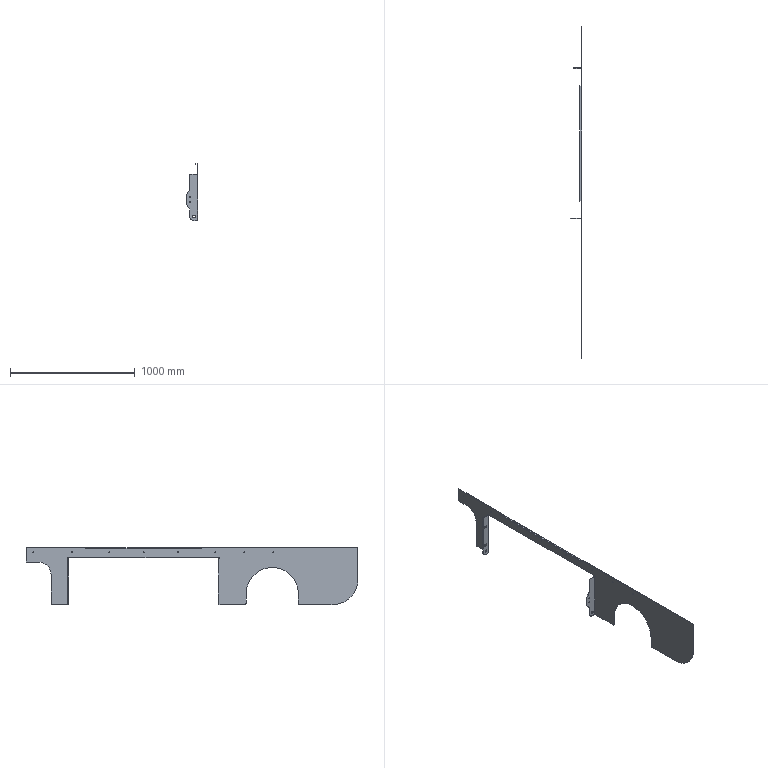Component | SolidWorks | BodySidePlate,Right-1 | 1 solid | 97 faces | volume 3195637 mm3 | plane 55 | cylinder 42 | commonest cylinder face diameters 7.2 x16 10.2 x4 20.2 x4 10 x4 20 x3 2 x3 12 x3 66 x2 | material Q235